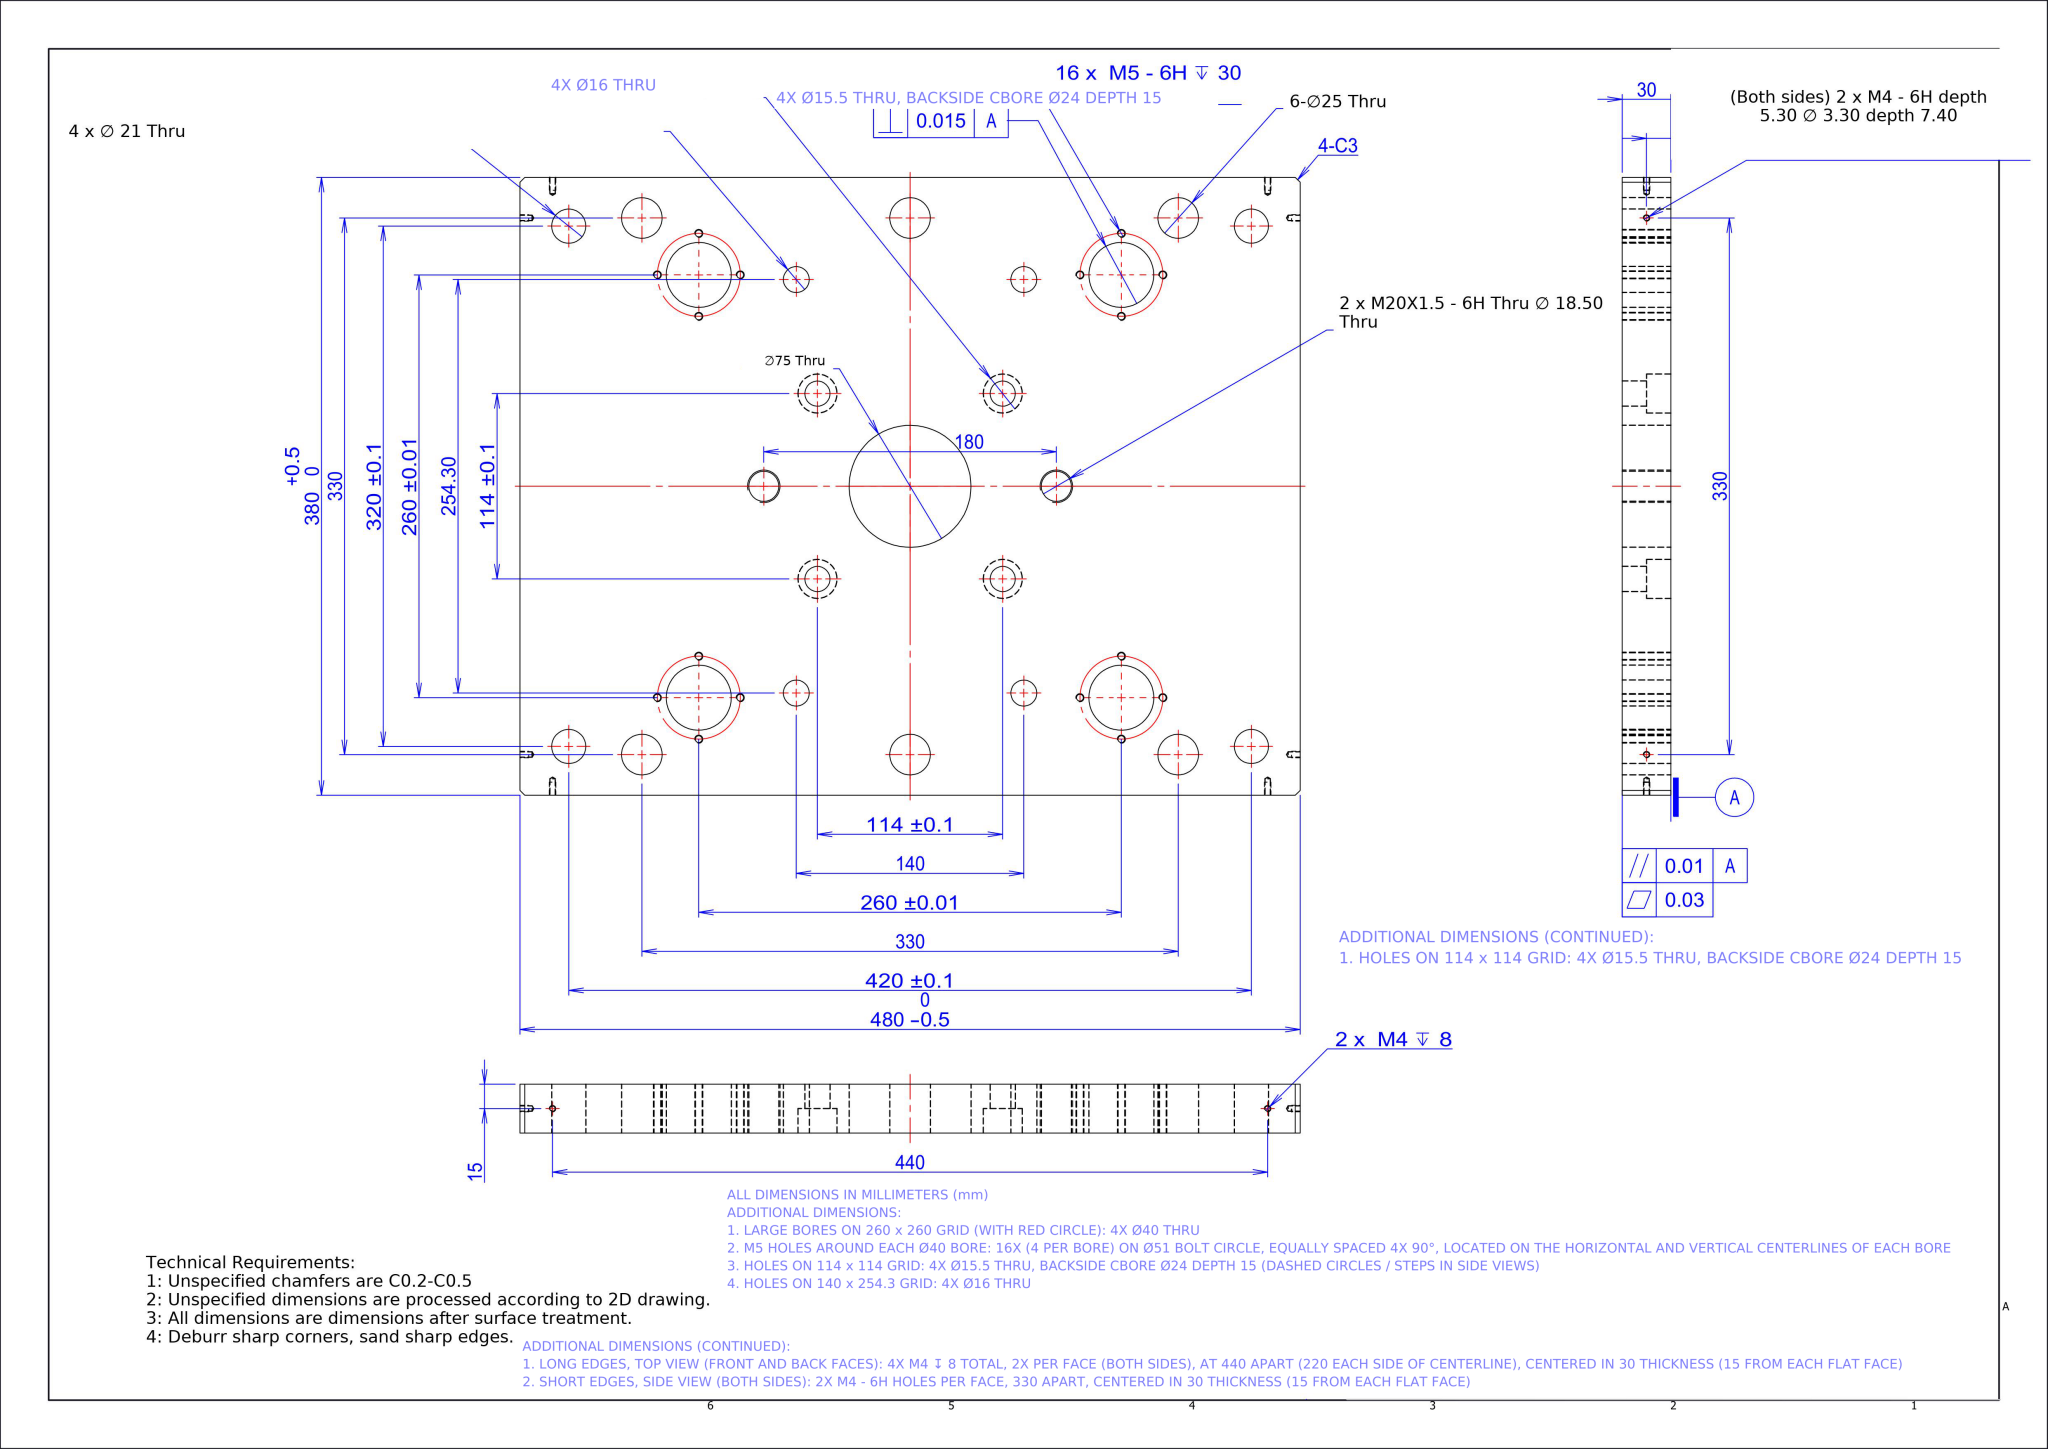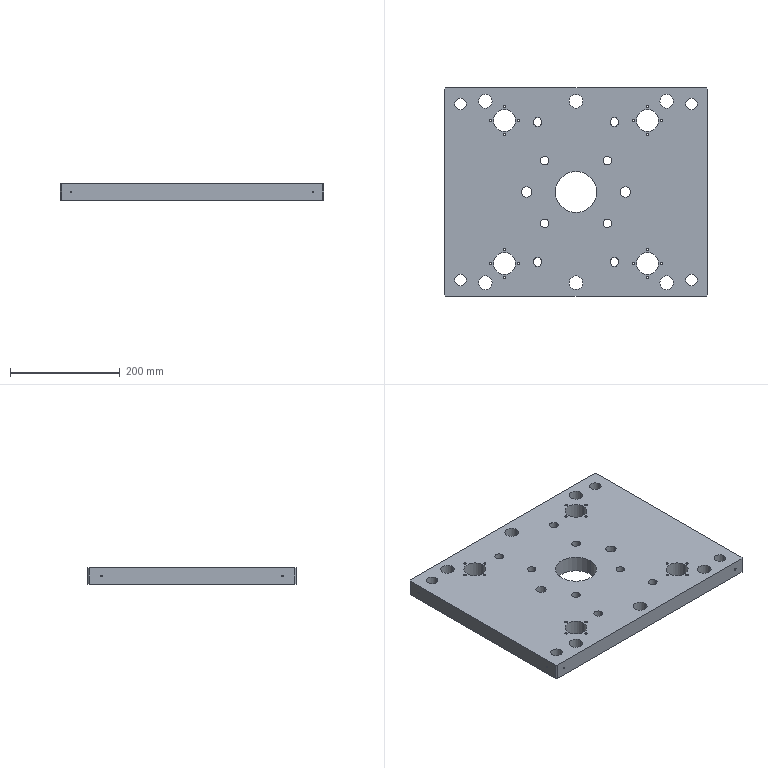Part | NX | mm | 1 solid | 136 faces | box 480 x 380 x 30 mm | volume 4972215 mm3 | cylinder 106 | cone 16 | plane 14 | commonest cylinder face diameters 4.2 x32 3.3 x16 25 x12 40 x8 16 x8 24 x8 15.5 x8 21 x8